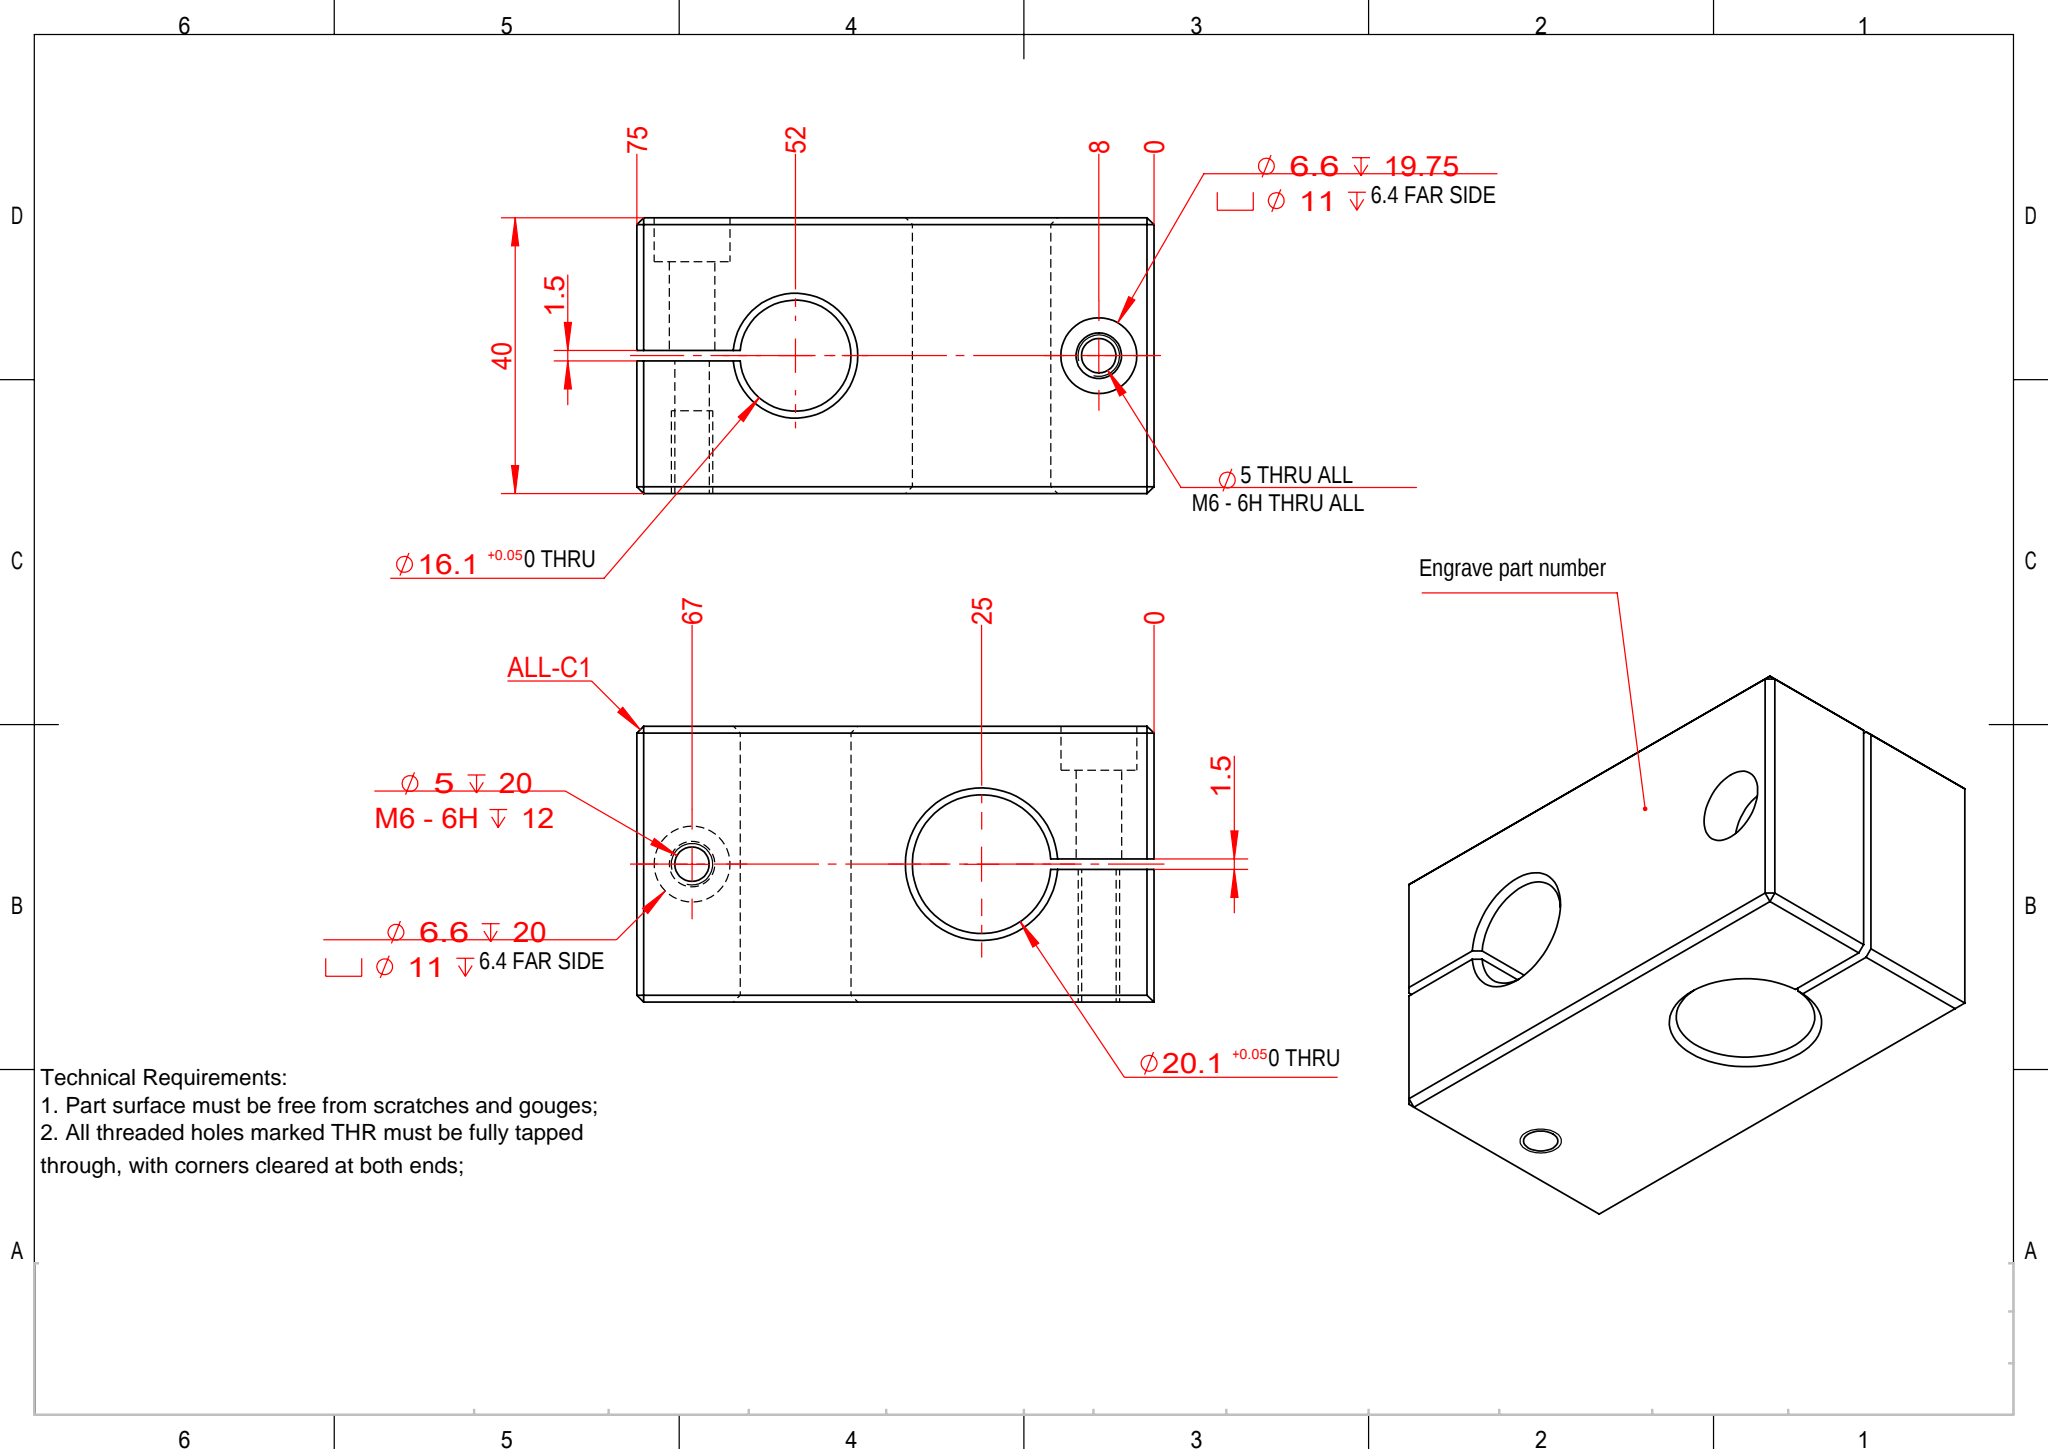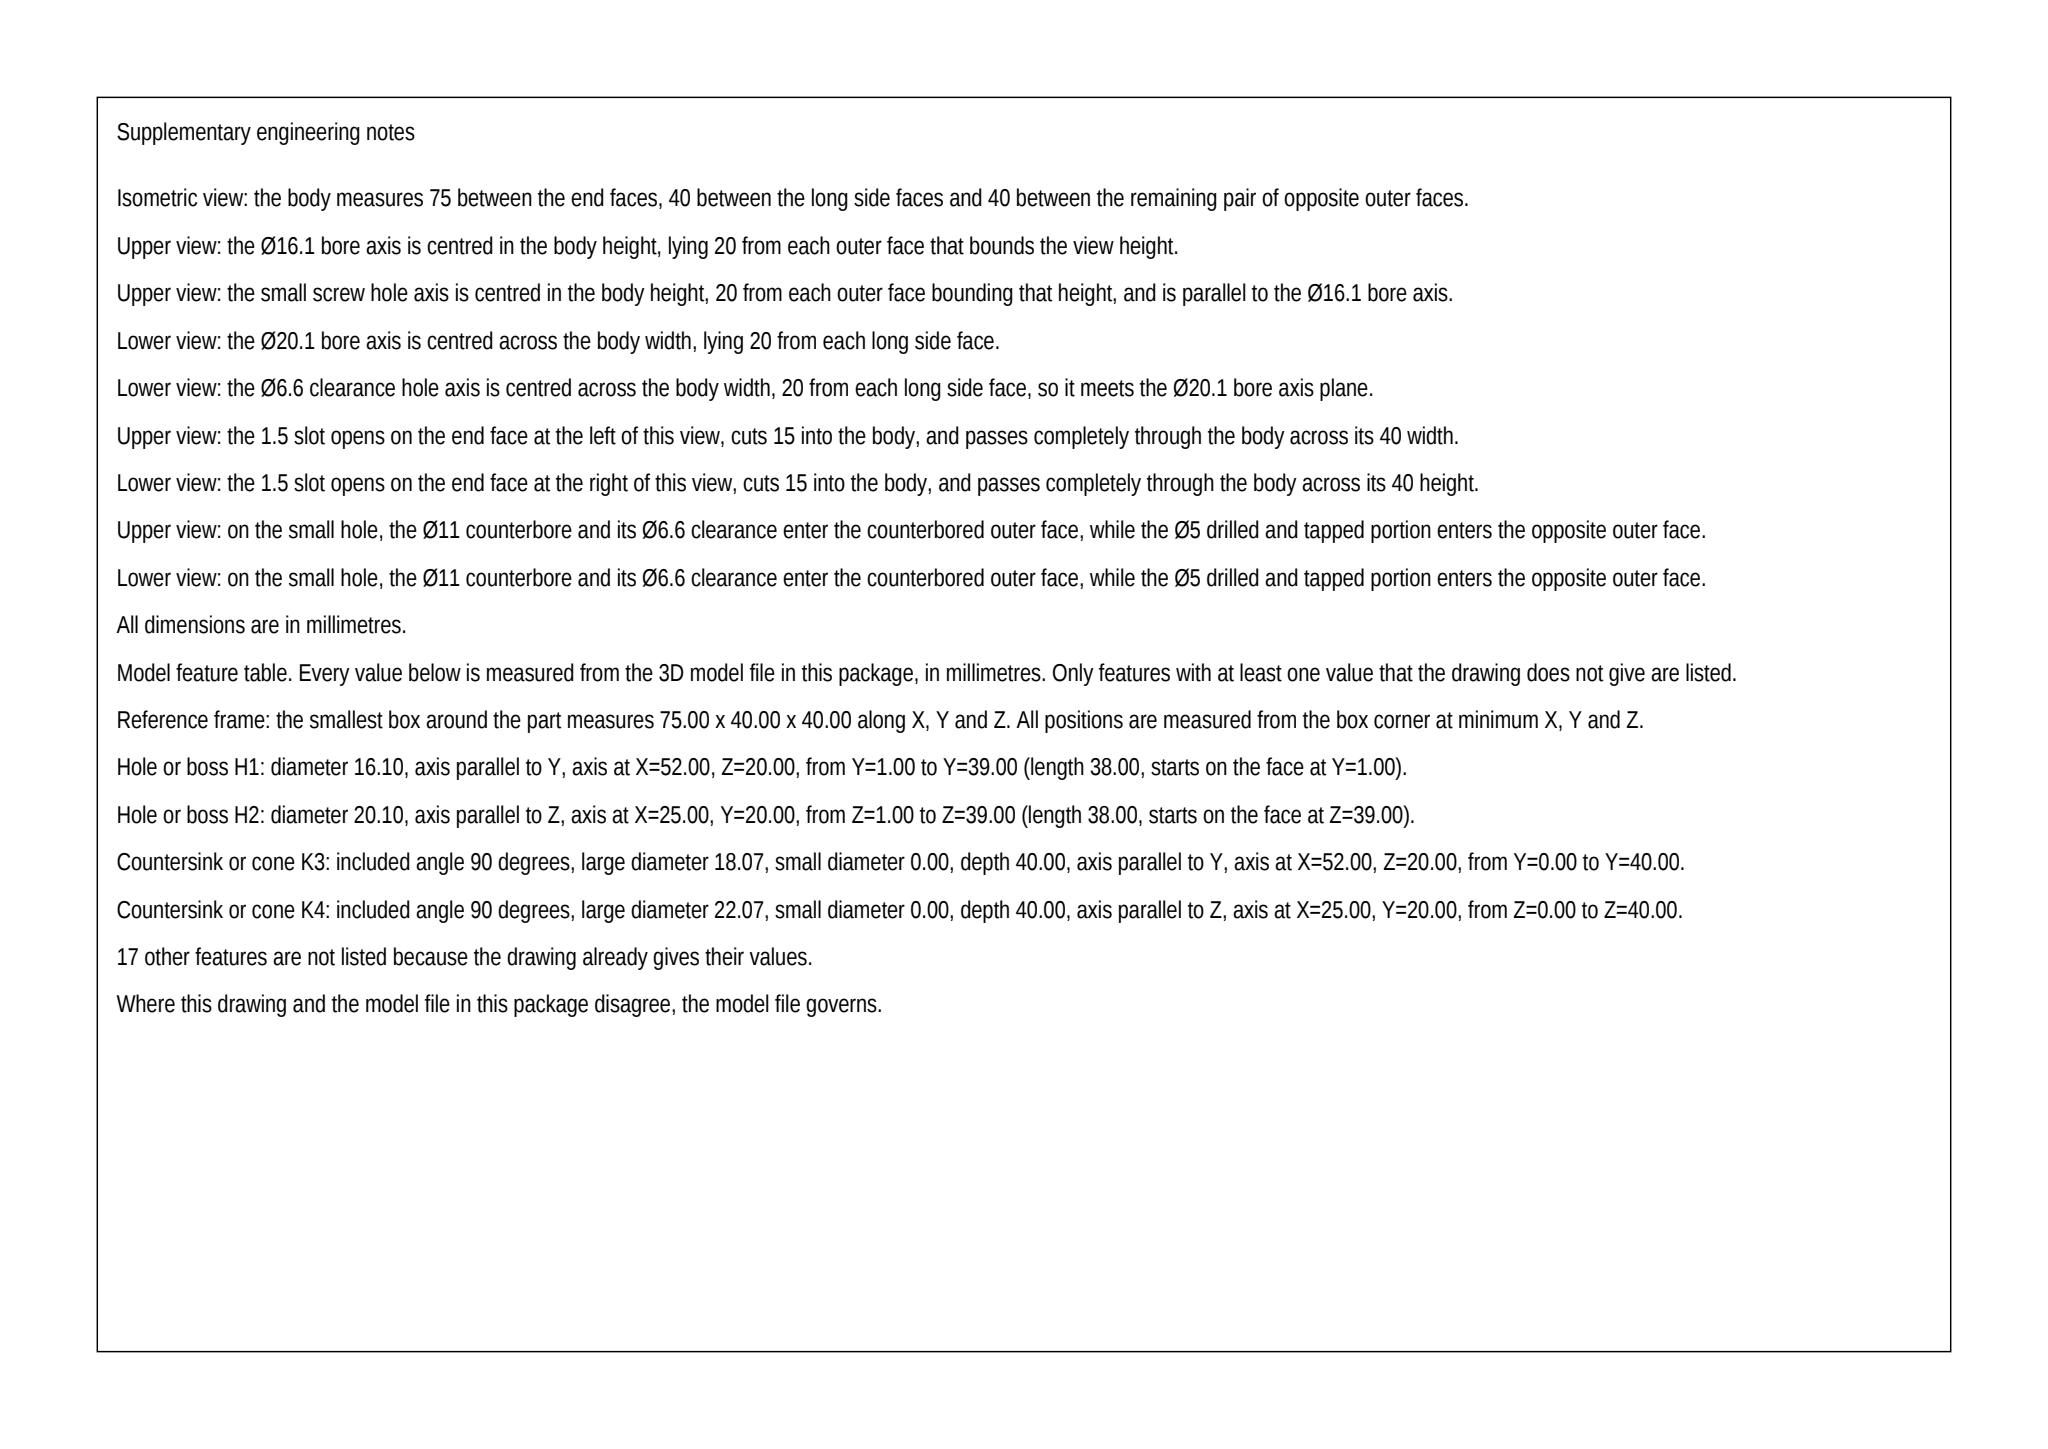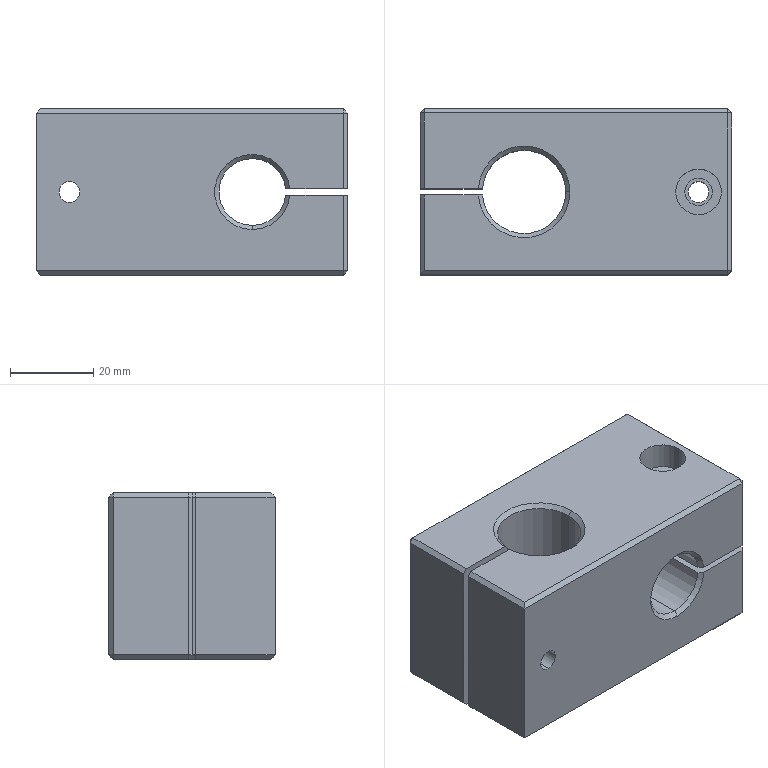Part | SolidWorks | mm | 1 solid | 61 faces | box 75 x 40 x 40 mm | volume 94120 mm3 | plane 35 | cylinder 17 | cone 9 | commonest cylinder face diameters 5 x4 6.6 x4 11 x4 16.1 x3 20.1 x2
Drawing notes:
TOP VIEW: OVERALL DEPTH (Y) 40 FROM FRONT FACE TO BACK FACE | from the solid: bbox_xyz Y=40.0; y-normal planes at 0.0 and 40.0
FRONT VIEW: Ø16.1, Ø6.6/Ø11/M6 & 1.5 SLOT AXES 20 FROM BOTTOM FACE | from the solid: Cyl dia16.1 axis y at z=20; dia6.6/11/5 axis y at x=8,z=20; slot faces y-planes 19.25 & 20.75 (1.5 wide ctr 20); bbox Z=40
TOP VIEW: Ø20.1, Ø5/Ø6.6/Ø11/M6 & 1.5 SLOT AXES 20 FROM FRONT FACE | from the solid: Cyl dia20.1 axis z at y=20; dia5/6.6/11 axis z at x=67,y=20; slot faces z-planes 19.25 & 20.75 (1.5 wide ctr 20); bbox Y=40
build123d program:
from build123d import *

# Parameters (mm, degrees)
SKETCH1_W                                       = 75
SKETCH1_H                                       = 40
BOSS_EXTRUDE1_DEPTH                             = 40
SKETCH2_R                                       = 10.05
CUT_EXTRUDE1_DEPTH                              = 94.941
SKETCH3_W                                       = 15
SKETCH3_H                                       = 1.5
CUT_EXTRUDE2_DEPTH                              = 94.941
CHAMFER1_SIZE                                   = 1
M6_HEX_SOCKET_HEAD_CAP_SCREW_CBORE1_D           = 6.6
M6_HEX_SOCKET_HEAD_CAP_SCREW_CBORE1_DEPTH       = 19.75
M6_HEX_SOCKET_HEAD_CAP_SCREW_CBORE1_CBORE_D     = 11
M6_HEX_SOCKET_HEAD_CAP_SCREW_CBORE1_CBORE_DEPTH = 6.4
M6_HEX_SOCKET_HEAD_CAP_SCREW_CBORE1_TIP         = 1.983
M6_TAPPED_HOLE1_D                               = 5
SKETCH10_R                                      = 8.05
CUT_EXTRUDE3_DEPTH                              = 94.941
CHAMFER2_SIZE                                   = 1
SKETCH11_W                                      = 15
SKETCH11_H                                      = 1.5
CUT_EXTRUDE4_DEPTH                              = 94.941
M6_HEX_SOCKET_HEAD_CAP_SCREW_CBORE2_D           = 6.6
M6_HEX_SOCKET_HEAD_CAP_SCREW_CBORE2_DEPTH       = 20
M6_HEX_SOCKET_HEAD_CAP_SCREW_CBORE2_CBORE_D     = 11
M6_HEX_SOCKET_HEAD_CAP_SCREW_CBORE2_CBORE_DEPTH = 6.4
M6_HEX_SOCKET_HEAD_CAP_SCREW_CBORE2_TIP         = 1.983
M6_TAPPED_HOLE2_D                               = 5
M6_TAPPED_HOLE2_DEPTH                           = 20
M6_TAPPED_HOLE2_TIP                             = 1.502
CHAMFER3_SIZE                                   = 1


with BuildPart() as part:
    # Sketch1 → Boss-Extrude1 (new body)
    with BuildSketch(Plane.XY):
        with Locations((37.5, 20)):
            Rectangle(SKETCH1_W, SKETCH1_H)
    extrude(amount=BOSS_EXTRUDE1_DEPTH)

    # Sketch2 → Cut-Extrude1 (cut, through all)
    with BuildSketch(Plane.XY.offset(40)):
        with Locations((25, 20)):
            Circle(SKETCH2_R)
    extrude(amount=-CUT_EXTRUDE1_DEPTH, mode=Mode.SUBTRACT)

    # Sketch3 → Cut-Extrude2 (cut, through all)
    with BuildSketch(Plane.XY.offset(40)):
        with Locations((7.5, 20)):
            Rectangle(SKETCH3_W, SKETCH3_H)
    extrude(amount=-CUT_EXTRUDE2_DEPTH, mode=Mode.SUBTRACT)

    # Chamfer1
    chamfer1_edges = [part.edges().sort_by_distance(p)[0] for p in [
        (25.375, 9.957, 0),
        (25.375, 9.957, 40),
    ]]
    chamfer(chamfer1_edges, length=CHAMFER1_SIZE)

    # M6 Hex Socket Head Cap Screw CBORE1
    with Locations(Plane(origin=(0, 40, 0), x_dir=(1, 0, 0), z_dir=(0, 1, 0))):
        with Locations((8, -20)):
            CounterBoreHole(M6_HEX_SOCKET_HEAD_CAP_SCREW_CBORE1_D / 2, M6_HEX_SOCKET_HEAD_CAP_SCREW_CBORE1_CBORE_D / 2, M6_HEX_SOCKET_HEAD_CAP_SCREW_CBORE1_CBORE_DEPTH, depth=M6_HEX_SOCKET_HEAD_CAP_SCREW_CBORE1_DEPTH)
            with Locations((0, 0, -(M6_HEX_SOCKET_HEAD_CAP_SCREW_CBORE1_DEPTH + M6_HEX_SOCKET_HEAD_CAP_SCREW_CBORE1_TIP / 2))):  # 118° drill point
                Cone(0, M6_HEX_SOCKET_HEAD_CAP_SCREW_CBORE1_D / 2, M6_HEX_SOCKET_HEAD_CAP_SCREW_CBORE1_TIP, mode=Mode.SUBTRACT)

    # M6 Tapped Hole1 (through all)
    with Locations(Plane(origin=(0, 0, 0), x_dir=(-1, 0, 0), z_dir=(0, -1, 0))):
        with Locations((-8, -20)):
            Hole(M6_TAPPED_HOLE1_D / 2)

    # Sketch10 → Cut-Extrude3 (cut, through all)
    with BuildSketch(Plane.XZ):
        with Locations(Location((52, 20, 0), (0, 0, 270))):
            Circle(SKETCH10_R)
    extrude(amount=-CUT_EXTRUDE3_DEPTH, mode=Mode.SUBTRACT)

    # Chamfer2
    chamfer2_edges = [part.edges().sort_by_distance(p)[0] for p in [
        (52, 40, 28.05),
        (52, 0, 28.05),
    ]]
    chamfer(chamfer2_edges, length=CHAMFER2_SIZE)

    # Sketch11 → Cut-Extrude4 (cut, through all)
    with BuildSketch(Plane.XZ):
        with Locations((67.5, 20)):
            Rectangle(SKETCH11_W, SKETCH11_H)
    extrude(amount=-CUT_EXTRUDE4_DEPTH, mode=Mode.SUBTRACT)

    # M6 Hex Socket Head Cap Screw CBORE2
    with Locations(Plane.XY.offset(40)):
        with Locations((67, 20)):
            CounterBoreHole(M6_HEX_SOCKET_HEAD_CAP_SCREW_CBORE2_D / 2, M6_HEX_SOCKET_HEAD_CAP_SCREW_CBORE2_CBORE_D / 2, M6_HEX_SOCKET_HEAD_CAP_SCREW_CBORE2_CBORE_DEPTH, depth=M6_HEX_SOCKET_HEAD_CAP_SCREW_CBORE2_DEPTH)
            with Locations((0, 0, -(M6_HEX_SOCKET_HEAD_CAP_SCREW_CBORE2_DEPTH + M6_HEX_SOCKET_HEAD_CAP_SCREW_CBORE2_TIP / 2))):  # 118° drill point
                Cone(0, M6_HEX_SOCKET_HEAD_CAP_SCREW_CBORE2_D / 2, M6_HEX_SOCKET_HEAD_CAP_SCREW_CBORE2_TIP, mode=Mode.SUBTRACT)

    # M6 Tapped Hole2
    with Locations(Plane(origin=(0, 0, 0), x_dir=(-1, 0, 0), z_dir=(0, 0, -1))):
        with Locations((-67, 20)):
            Hole(M6_TAPPED_HOLE2_D / 2, depth=M6_TAPPED_HOLE2_DEPTH)
            with Locations((0, 0, -(M6_TAPPED_HOLE2_DEPTH + M6_TAPPED_HOLE2_TIP / 2))):  # 118° drill point
                Cone(0, M6_TAPPED_HOLE2_D / 2, M6_TAPPED_HOLE2_TIP, mode=Mode.SUBTRACT)

    # Chamfer3
    chamfer3_edges = [part.edges().sort_by_distance(p)[0] for p in [
        (75, 20, 40),
        (37.5, 40, 40),
        (0, 9.625, 0),
        (0, 9.625, 40),
        (0, 30.375, 40),
        (37.5, 40, 0),
        (75, 20, 0),
        (37.5, 0, 0),
        (0, 30.375, 0),
        (37.5, 0, 40),
        (0, 40, 20),
        (75, 40, 30.375),
        (75, 0, 30.375),
        (75, 40, 9.625),
        (75, 0, 9.625),
    ]]
    chamfer(chamfer3_edges, length=CHAMFER3_SIZE)


solid = part.part